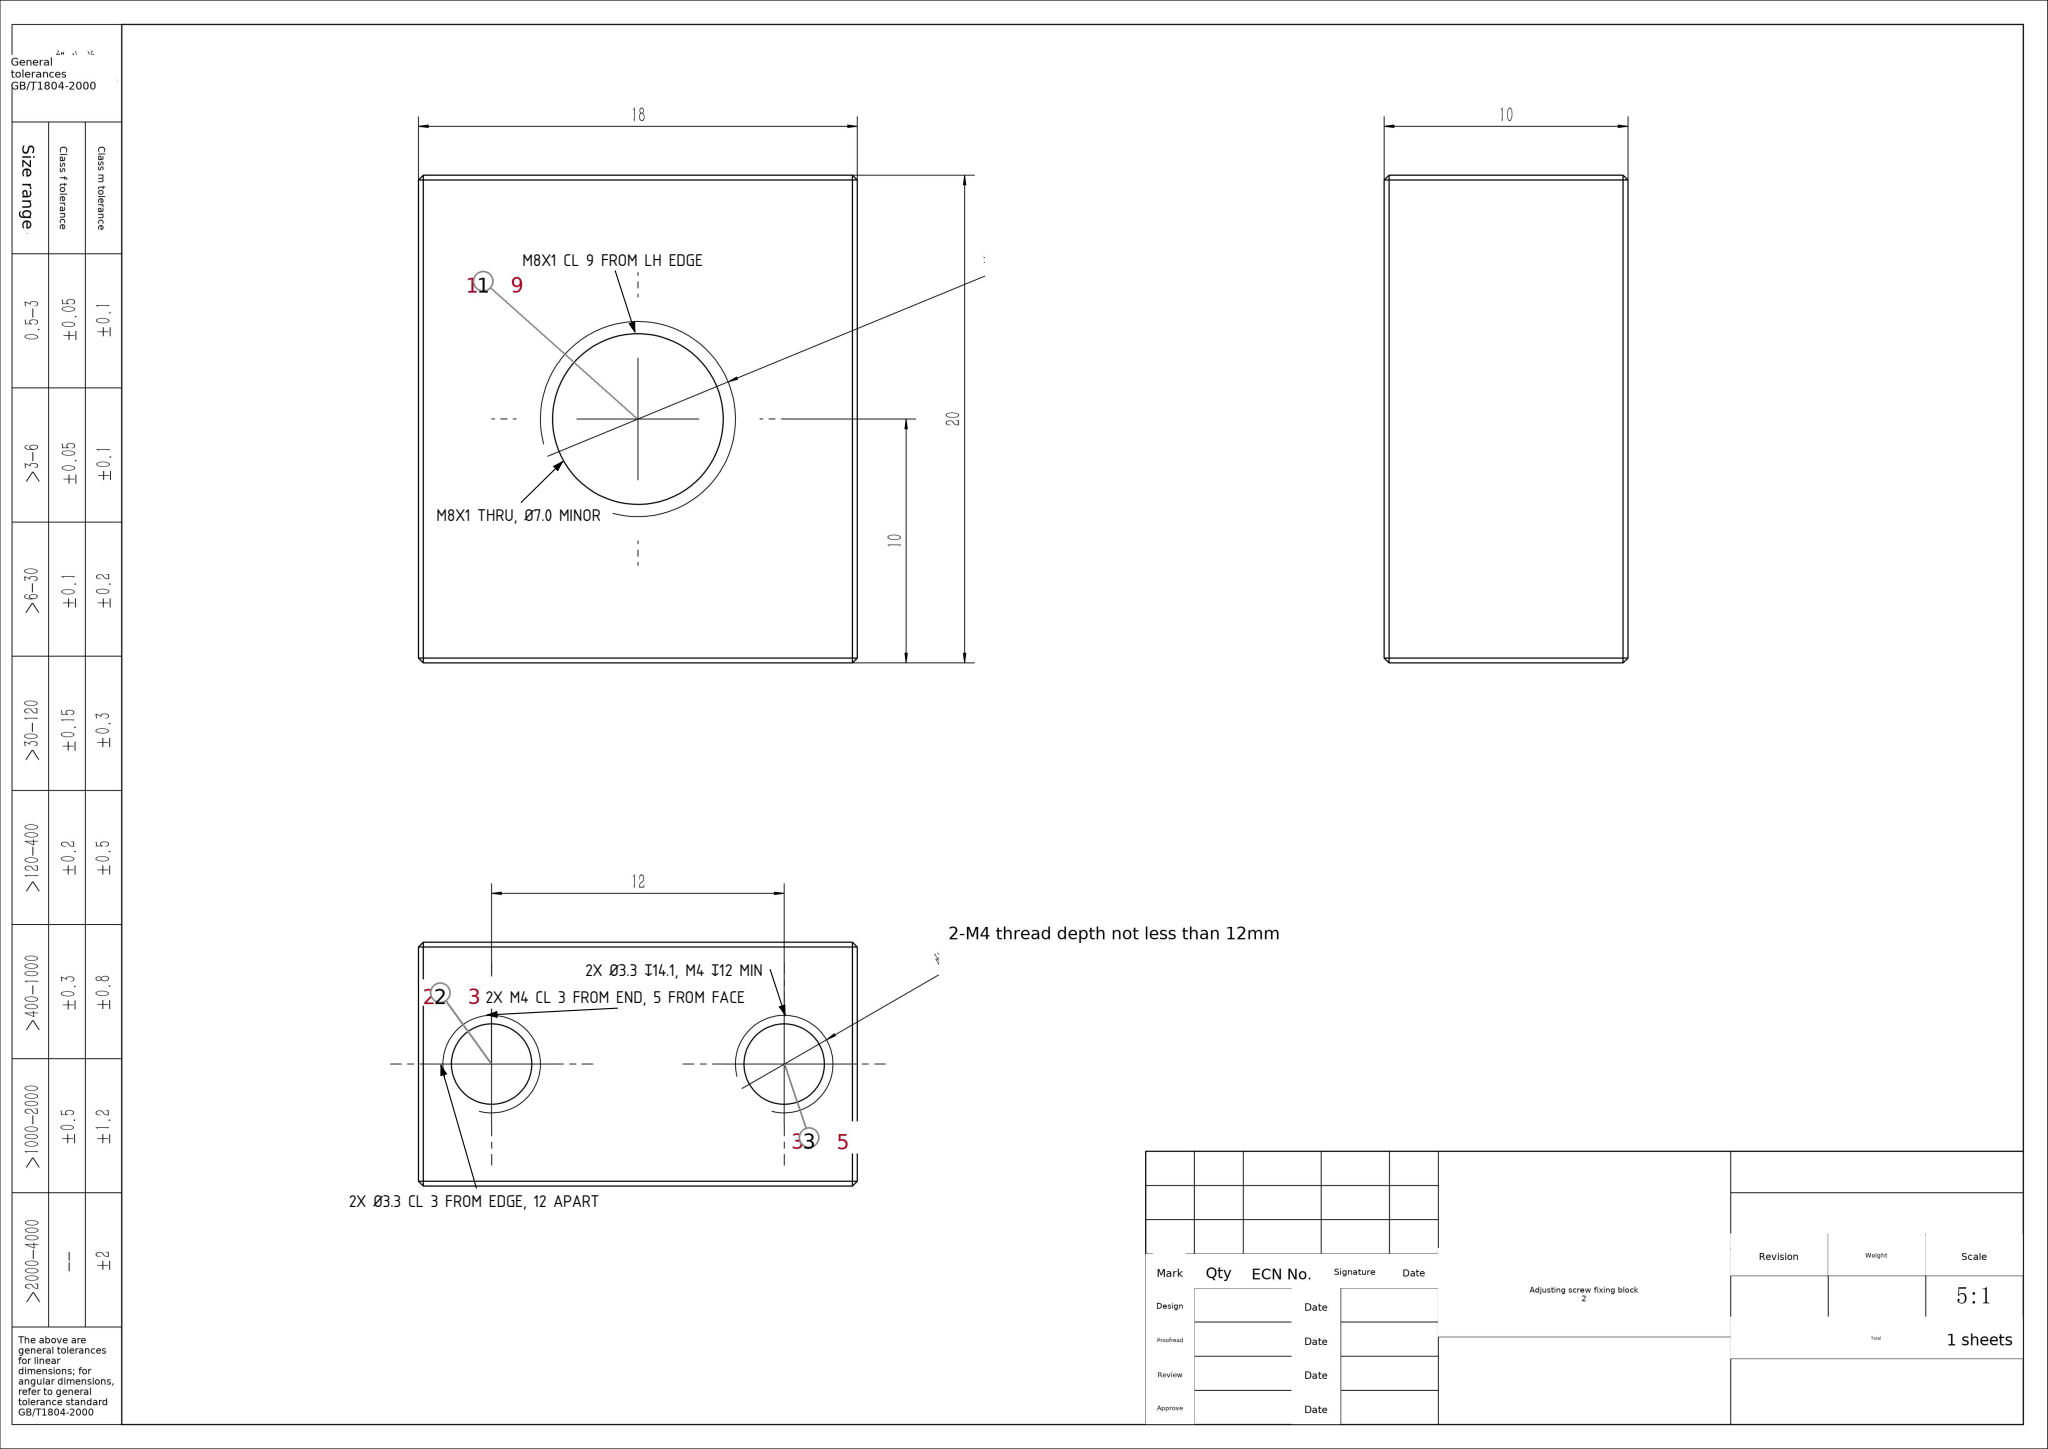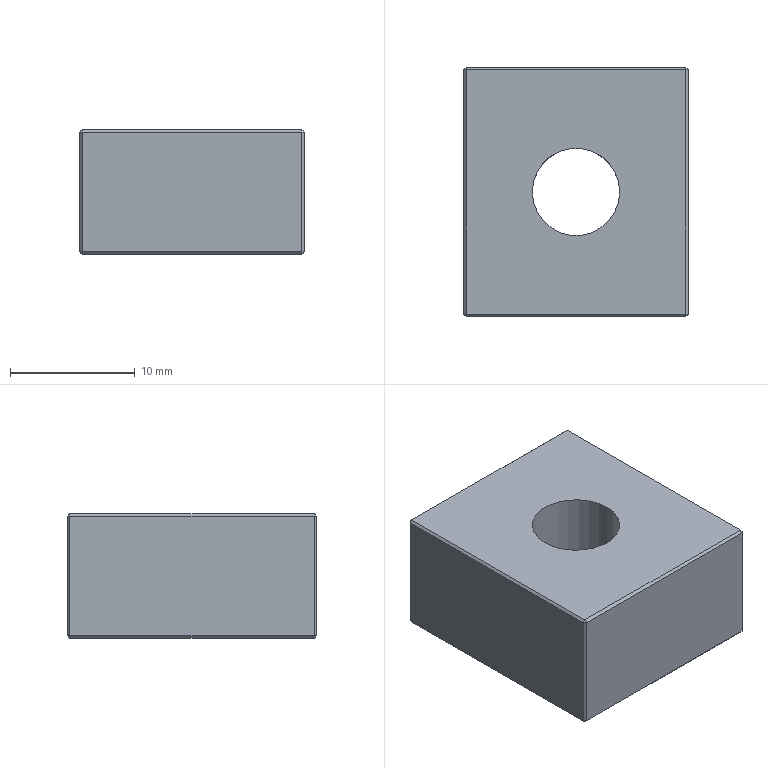Part | SolidWorks | mm | 1 solid | 36 faces | box 18 x 20 x 10 mm | volume 2965 mm3 | plane 26 | cylinder 6 | cone 4 | commonest cylinder face diameters 3.3 x4 7 x2
Drawing notes:
M8X1 HOLE CL 9 FROM LH EDGE (CENTERED IN 18 WIDTH) | from the solid: Ø7.0 z-axis cyl at x=9.0 of 18.0 bbox width
2X M4 HOLE CL 3 FROM EACH END, 5 FROM FACE (CTR OF 10 THK) | from the solid: Ø3.3 y-axis cyls at x=3.0 & 15.0, z=5.0; bbox 18x20x10
2X Ø3.3 DRILL DP 14.1 (118° PT), M4 DP 12 MIN | from the solid: Ø3.3 y-axis cyl length 14.1, cone incl angle 118° ref dia 3.3
CTR HOLE: M8X1 THRU, Ø7.0 MINOR DIA, FULL THD 10 DEEP | from the solid: Ø7.0 cyl, axis Z, pos (9.0,10.0), length 10.0 = full 10 thk; minor dia 7.0 -> M8x1 fine
2X Ø3.3 M4 THD: CL 3.0 FROM LH EDGE, 12 APART, 5.0 FROM FACE | from the solid: Ø3.3 cyls axis Y at x=3.0 and x=15.0, z=5.0; bbox X=18.0 so 15.0 = 3.0 from RH edge
build123d program:
from build123d import *

# Parameters (mm, degrees)
SKETCH1_W             = 18
SKETCH1_H             = 10
BOSS_EXTRUDE1_DEPTH   = 10
M4_TAPPED_HOLE1_D     = 3.3
M4_TAPPED_HOLE1_DEPTH = 14.1
M4_TAPPED_HOLE1_TIP   = 0.9914
M8X1_0_TAPPED_HOLE1_D = 7
CHAMFER1_SIZE         = 0.2


with BuildPart() as part:
    # Sketch1 → Boss-Extrude1 (new, symmetric)
    with BuildSketch(Plane(origin=(0, 0, 0), x_dir=(1, 0, 0), z_dir=(0, 1, 0))):
        Rectangle(SKETCH1_W, SKETCH1_H)
    extrude(amount=BOSS_EXTRUDE1_DEPTH, both=True)

    # M4 Tapped Hole1
    with Locations(Plane(origin=(0, 10, 0), x_dir=(1, 0, 0), z_dir=(0, 1, 0))):
        with Locations((-6, 0), (6, 0)):
            Hole(M4_TAPPED_HOLE1_D / 2, depth=M4_TAPPED_HOLE1_DEPTH)
            with Locations((0, 0, -(M4_TAPPED_HOLE1_DEPTH + M4_TAPPED_HOLE1_TIP / 2))):  # 118° drill point
                Cone(0, M4_TAPPED_HOLE1_D / 2, M4_TAPPED_HOLE1_TIP, mode=Mode.SUBTRACT)

    # M8x1.0 Tapped Hole1 (through all)
    with Locations(Plane.XY.offset(5)):
        with Locations((0, 0)):
            Hole(M8X1_0_TAPPED_HOLE1_D / 2)

    # Chamfer1
    chamfer1_edges = [part.edges().sort_by_distance(p)[0] for p in [
        (-9, 10, 0),
        (0, 10, 5),
        (9, 10, 0),
        (0, -10, 5),
        (-9, -10, 0),
        (0, -10, -5),
        (9, -10, 0),
        (9, 0, 5),
        (-9, 0, 5),
        (-9, 0, -5),
        (9, 0, -5),
        (0, 10, -5),
    ]]
    chamfer(chamfer1_edges, length=CHAMFER1_SIZE)


solid = part.part
STEP:
#1=CARTESIAN_POINT('',(-3.5,0.,-5.));
#2=VERTEX_POINT('',#1);
#3=CARTESIAN_POINT('',(3.5,0.,-5.));
#4=VERTEX_POINT('',#3);
#5=CARTESIAN_POINT('',(0.,0.,-5.));
#6=DIRECTION('',(0.,0.,1.));
#7=DIRECTION('',(1.,0.,0.));
#8=AXIS2_PLACEMENT_3D('',#5,#6,#7);
#9=CIRCLE('',#8,3.5);
#10=EDGE_CURVE('',#2,#4,#9,.T.);
#11=ORIENTED_EDGE('',*,*,#10,.F.);
#12=CARTESIAN_POINT('',(-3.5,0.,5.));
#13=VERTEX_POINT('',#12);
#14=CARTESIAN_POINT('',(-3.5,0.,5.));
#15=DIRECTION('',(0.,0.,1.));
#16=VECTOR('',#15,1000.);
#17=LINE('',#14,#16);
#18=EDGE_CURVE('',#2,#13,#17,.T.);
#19=ORIENTED_EDGE('',*,*,#18,.T.);
#20=CARTESIAN_POINT('',(3.5,0.,5.));
#21=VERTEX_POINT('',#20);
#22=CARTESIAN_POINT('',(0.,0.,5.));
#23=DIRECTION('',(0.,0.,1.));
#24=DIRECTION('',(1.,0.,0.));
#25=AXIS2_PLACEMENT_3D('',#22,#23,#24);
#26=CIRCLE('',#25,3.5);
#27=EDGE_CURVE('',#13,#21,#26,.T.);
#28=ORIENTED_EDGE('',*,*,#27,.T.);
#29=CARTESIAN_POINT('',(3.5,0.,5.));
#30=DIRECTION('',(0.,0.,1.));
#31=VECTOR('',#30,1000.);
#32=LINE('',#29,#31);
#33=EDGE_CURVE('',#4,#21,#32,.T.);
#34=ORIENTED_EDGE('',*,*,#33,.F.);
#35=EDGE_LOOP('',(#11,#19,#28,#34));
#36=FACE_OUTER_BOUND('',#35,.T.);
#37=CARTESIAN_POINT('',(0.,0.,5.));
#38=DIRECTION('',(0.,0.,1.));
#39=DIRECTION('',(1.,0.,0.));
#40=AXIS2_PLACEMENT_3D('',#37,#38,#39);
#41=CYLINDRICAL_SURFACE('',#40,3.5);
#42=ADVANCED_FACE('',(#36),#41,.F.);
#43=CARTESIAN_POINT('',(-6.,-4.1,-1.65));
#44=VERTEX_POINT('',#43);
#45=CARTESIAN_POINT('',(-6.,-4.1,1.65));
#46=VERTEX_POINT('',#45);
#47=CARTESIAN_POINT('',(-6.,-4.1,0.));
#48=DIRECTION('',(0.,1.,0.));
#49=DIRECTION('',(0.,0.,1.));
#50=AXIS2_PLACEMENT_3D('',#47,#48,#49);
#51=CIRCLE('',#50,1.65);
#52=EDGE_CURVE('',#44,#46,#51,.T.);
#53=ORIENTED_EDGE('',*,*,#52,.F.);
#54=CARTESIAN_POINT('',(-6.,10.,-1.65));
#55=VERTEX_POINT('',#54);
#56=CARTESIAN_POINT('',(-6.,10.,-1.65));
#57=DIRECTION('',(0.,1.,0.));
#58=VECTOR('',#57,1000.);
#59=LINE('',#56,#58);
#60=EDGE_CURVE('',#44,#55,#59,.T.);
#61=ORIENTED_EDGE('',*,*,#60,.T.);
#62=CARTESIAN_POINT('',(-6.,10.,1.65));
#63=VERTEX_POINT('',#62);
#64=CARTESIAN_POINT('',(-6.,10.,0.));
#65=DIRECTION('',(0.,1.,0.));
#66=DIRECTION('',(0.,0.,1.));
#67=AXIS2_PLACEMENT_3D('',#64,#65,#66);
#68=CIRCLE('',#67,1.65);
#69=EDGE_CURVE('',#55,#63,#68,.T.);
#70=ORIENTED_EDGE('',*,*,#69,.T.);
#71=CARTESIAN_POINT('',(-6.,10.,1.65));
#72=DIRECTION('',(0.,1.,0.));
#73=VECTOR('',#72,1000.);
#74=LINE('',#71,#73);
#75=EDGE_CURVE('',#46,#63,#74,.T.);
#76=ORIENTED_EDGE('',*,*,#75,.F.);
#77=EDGE_LOOP('',(#53,#61,#70,#76));
#78=FACE_OUTER_BOUND('',#77,.T.);
#79=CARTESIAN_POINT('',(-6.,10.,0.));
#80=DIRECTION('',(0.,1.,0.));
#81=DIRECTION('',(0.,0.,1.));
#82=AXIS2_PLACEMENT_3D('',#79,#80,#81);
#83=CYLINDRICAL_SURFACE('',#82,1.65);
#84=ADVANCED_FACE('',(#78),#83,.F.);
#85=CARTESIAN_POINT('',(-6.,-5.091,0.));
#86=VERTEX_POINT('',#85);
#87=CARTESIAN_POINT('',(-6.,-4.1,1.65));
#88=DIRECTION('',(0.,0.515,0.8572));
#89=VECTOR('',#88,1000.);
#90=LINE('',#87,#89);
#91=EDGE_CURVE('',#86,#46,#90,.T.);
#92=ORIENTED_EDGE('',*,*,#91,.F.);
#93=CARTESIAN_POINT('',(-6.,-4.1,-1.65));
#94=DIRECTION('',(0.,0.515,-0.8572));
#95=VECTOR('',#94,1000.);
#96=LINE('',#93,#95);
#97=EDGE_CURVE('',#86,#44,#96,.T.);
#98=ORIENTED_EDGE('',*,*,#97,.T.);
#99=ORIENTED_EDGE('',*,*,#52,.T.);
#100=EDGE_LOOP('',(#92,#98,#99));
#101=FACE_OUTER_BOUND('',#100,.T.);
#102=CARTESIAN_POINT('',(-6.,-4.1,0.));
#103=DIRECTION('',(0.,1.,0.));
#104=DIRECTION('',(0.,0.,1.));
#105=AXIS2_PLACEMENT_3D('',#102,#103,#104);
#106=CONICAL_SURFACE('',#105,1.65,1.03);
#107=ADVANCED_FACE('',(#101),#106,.F.);
#108=CARTESIAN_POINT('',(6.,-4.1,-1.65));
#109=VERTEX_POINT('',#108);
#110=CARTESIAN_POINT('',(6.,-4.1,1.65));
#111=VERTEX_POINT('',#110);
#112=CARTESIAN_POINT('',(6.,-4.1,-0.));
#113=DIRECTION('',(0.,1.,0.));
#114=DIRECTION('',(0.,0.,1.));
#115=AXIS2_PLACEMENT_3D('',#112,#113,#114);
#116=CIRCLE('',#115,1.65);
#117=EDGE_CURVE('',#109,#111,#116,.T.);
#118=ORIENTED_EDGE('',*,*,#117,.F.);
#119=CARTESIAN_POINT('',(6.,10.,-1.65));
#120=VERTEX_POINT('',#119);
#121=CARTESIAN_POINT('',(6.,10.,-1.65));
#122=DIRECTION('',(0.,1.,0.));
#123=VECTOR('',#122,1000.);
#124=LINE('',#121,#123);
#125=EDGE_CURVE('',#109,#120,#124,.T.);
#126=ORIENTED_EDGE('',*,*,#125,.T.);
#127=CARTESIAN_POINT('',(6.,10.,1.65));
#128=VERTEX_POINT('',#127);
#129=CARTESIAN_POINT('',(6.,10.,-0.));
#130=DIRECTION('',(0.,1.,0.));
#131=DIRECTION('',(0.,0.,1.));
#132=AXIS2_PLACEMENT_3D('',#129,#130,#131);
#133=CIRCLE('',#132,1.65);
#134=EDGE_CURVE('',#120,#128,#133,.T.);
#135=ORIENTED_EDGE('',*,*,#134,.T.);
#136=CARTESIAN_POINT('',(6.,10.,1.65));
#137=DIRECTION('',(0.,1.,0.));
#138=VECTOR('',#137,1000.);
#139=LINE('',#136,#138);
#140=EDGE_CURVE('',#111,#128,#139,.T.);
#141=ORIENTED_EDGE('',*,*,#140,.F.);
#142=EDGE_LOOP('',(#118,#126,#135,#141));
#143=FACE_OUTER_BOUND('',#142,.T.);
#144=CARTESIAN_POINT('',(6.,10.,-0.));
#145=DIRECTION('',(0.,1.,0.));
#146=DIRECTION('',(0.,0.,1.));
#147=AXIS2_PLACEMENT_3D('',#144,#145,#146);
#148=CYLINDRICAL_SURFACE('',#147,1.65);
#149=ADVANCED_FACE('',(#143),#148,.F.);
#150=CARTESIAN_POINT('',(6.,-5.091,-0.));
#151=VERTEX_POINT('',#150);
#152=CARTESIAN_POINT('',(6.,-4.1,1.65));
#153=DIRECTION('',(0.,0.515,0.8572));
#154=VECTOR('',#153,1000.);
#155=LINE('',#152,#154);
#156=EDGE_CURVE('',#151,#111,#155,.T.);
#157=ORIENTED_EDGE('',*,*,#156,.F.);
#158=CARTESIAN_POINT('',(6.,-4.1,-1.65));
#159=DIRECTION('',(0.,0.515,-0.8572));
#160=VECTOR('',#159,1000.);
#161=LINE('',#158,#160);
#162=EDGE_CURVE('',#151,#109,#161,.T.);
#163=ORIENTED_EDGE('',*,*,#162,.T.);
#164=ORIENTED_EDGE('',*,*,#117,.T.);
#165=EDGE_LOOP('',(#157,#163,#164));
#166=FACE_OUTER_BOUND('',#165,.T.);
#167=CARTESIAN_POINT('',(6.,-4.1,-0.));
#168=DIRECTION('',(0.,1.,0.));
#169=DIRECTION('',(0.,0.,1.));
#170=AXIS2_PLACEMENT_3D('',#167,#168,#169);
#171=CONICAL_SURFACE('',#170,1.65,1.03);
#172=ADVANCED_FACE('',(#166),#171,.F.);
#173=CARTESIAN_POINT('',(9.,9.8,-4.8));
#174=VERTEX_POINT('',#173);
#175=CARTESIAN_POINT('',(9.,9.8,4.8));
#176=VERTEX_POINT('',#175);
#177=CARTESIAN_POINT('',(9.,9.8,5.));
#178=DIRECTION('',(0.,0.,1.));
#179=VECTOR('',#178,1000.);
#180=LINE('',#177,#179);
#181=EDGE_CURVE('',#174,#176,#180,.T.);
#182=ORIENTED_EDGE('',*,*,#181,.T.);
#183=CARTESIAN_POINT('',(9.,-9.8,4.8));
#184=VERTEX_POINT('',#183);
#185=CARTESIAN_POINT('',(9.,10.,4.8));
#186=DIRECTION('',(0.,-1.,0.));
#187=VECTOR('',#186,1000.);
#188=LINE('',#185,#187);
#189=EDGE_CURVE('',#176,#184,#188,.T.);
#190=ORIENTED_EDGE('',*,*,#189,.T.);
#191=CARTESIAN_POINT('',(9.,-9.8,-4.8));
#192=VERTEX_POINT('',#191);
#193=CARTESIAN_POINT('',(9.,-9.8,-5.));
#194=DIRECTION('',(0.,0.,-1.));
#195=VECTOR('',#194,1000.);
#196=LINE('',#193,#195);
#197=EDGE_CURVE('',#184,#192,#196,.T.);
#198=ORIENTED_EDGE('',*,*,#197,.T.);
#199=CARTESIAN_POINT('',(9.,10.,-4.8));
#200=DIRECTION('',(0.,1.,0.));
#201=VECTOR('',#200,1000.);
#202=LINE('',#199,#201);
#203=EDGE_CURVE('',#192,#174,#202,.T.);
#204=ORIENTED_EDGE('',*,*,#203,.T.);
#205=EDGE_LOOP('',(#182,#190,#198,#204));
#206=FACE_OUTER_BOUND('',#205,.T.);
#207=CARTESIAN_POINT('',(9.,10.,-5.));
#208=DIRECTION('',(-1.,0.,0.));
#209=DIRECTION('',(0.,0.,1.));
#210=AXIS2_PLACEMENT_3D('',#207,#208,#209);
#211=PLANE('',#210);
#212=ADVANCED_FACE('',(#206),#211,.F.);
#213=CARTESIAN_POINT('',(8.8,-9.8,-5.));
#214=VERTEX_POINT('',#213);
#215=CARTESIAN_POINT('',(-8.8,-9.8,-5.));
#216=VERTEX_POINT('',#215);
#217=CARTESIAN_POINT('',(-9.,-9.8,-5.));
#218=DIRECTION('',(-1.,0.,0.));
#219=VECTOR('',#218,1000.);
#220=LINE('',#217,#219);
#221=EDGE_CURVE('',#214,#216,#220,.T.);
#222=ORIENTED_EDGE('',*,*,#221,.T.);
#223=CARTESIAN_POINT('',(-8.8,9.8,-5.));
#224=VERTEX_POINT('',#223);
#225=CARTESIAN_POINT('',(-8.8,10.,-5.));
#226=DIRECTION('',(0.,1.,0.));
#227=VECTOR('',#226,1000.);
#228=LINE('',#225,#227);
#229=EDGE_CURVE('',#216,#224,#228,.T.);
#230=ORIENTED_EDGE('',*,*,#229,.T.);
#231=CARTESIAN_POINT('',(8.8,9.8,-5.));
#232=VERTEX_POINT('',#231);
#233=CARTESIAN_POINT('',(9.,9.8,-5.));
#234=DIRECTION('',(1.,0.,0.));
#235=VECTOR('',#234,1000.);
#236=LINE('',#233,#235);
#237=EDGE_CURVE('',#224,#232,#236,.T.);
#238=ORIENTED_EDGE('',*,*,#237,.T.);
#239=CARTESIAN_POINT('',(8.8,10.,-5.));
#240=DIRECTION('',(0.,-1.,0.));
#241=VECTOR('',#240,1000.);
#242=LINE('',#239,#241);
#243=EDGE_CURVE('',#232,#214,#242,.T.);
#244=ORIENTED_EDGE('',*,*,#243,.T.);
#245=EDGE_LOOP('',(#222,#230,#238,#244));
#246=FACE_OUTER_BOUND('',#245,.T.);
#247=CARTESIAN_POINT('',(0.,0.,-5.));
#248=DIRECTION('',(0.,0.,1.));
#249=DIRECTION('',(1.,0.,0.));
#250=AXIS2_PLACEMENT_3D('',#247,#248,#249);
#251=CIRCLE('',#250,3.5);
#252=EDGE_CURVE('',#4,#2,#251,.T.);
#253=ORIENTED_EDGE('',*,*,#252,.T.);
#254=ORIENTED_EDGE('',*,*,#10,.T.);
#255=EDGE_LOOP('',(#253,#254));
#256=FACE_BOUND('',#255,.T.);
#257=CARTESIAN_POINT('',(-9.,10.,-5.));
#258=DIRECTION('',(0.,0.,1.));
#259=DIRECTION('',(1.,0.,0.));
#260=AXIS2_PLACEMENT_3D('',#257,#258,#259);
#261=PLANE('',#260);
#262=ADVANCED_FACE('',(#246,#256),#261,.F.);
#263=CARTESIAN_POINT('',(-9.,9.8,4.8));
#264=VERTEX_POINT('',#263);
#265=CARTESIAN_POINT('',(-9.,9.8,-4.8));
#266=VERTEX_POINT('',#265);
#267=CARTESIAN_POINT('',(-9.,9.8,-5.));
#268=DIRECTION('',(0.,0.,-1.));
#269=VECTOR('',#268,1000.);
#270=LINE('',#267,#269);
#271=EDGE_CURVE('',#264,#266,#270,.T.);
#272=ORIENTED_EDGE('',*,*,#271,.T.);
#273=CARTESIAN_POINT('',(-9.,-9.8,-4.8));
#274=VERTEX_POINT('',#273);
#275=CARTESIAN_POINT('',(-9.,10.,-4.8));
#276=DIRECTION('',(0.,-1.,0.));
#277=VECTOR('',#276,1000.);
#278=LINE('',#275,#277);
#279=EDGE_CURVE('',#266,#274,#278,.T.);
#280=ORIENTED_EDGE('',*,*,#279,.T.);
#281=CARTESIAN_POINT('',(-9.,-9.8,4.8));
#282=VERTEX_POINT('',#281);
#283=CARTESIAN_POINT('',(-9.,-9.8,-5.));
#284=DIRECTION('',(0.,0.,1.));
#285=VECTOR('',#284,1000.);
#286=LINE('',#283,#285);
#287=EDGE_CURVE('',#274,#282,#286,.T.);
#288=ORIENTED_EDGE('',*,*,#287,.T.);
#289=CARTESIAN_POINT('',(-9.,10.,4.8));
#290=DIRECTION('',(0.,1.,0.));
#291=VECTOR('',#290,1000.);
#292=LINE('',#289,#291);
#293=EDGE_CURVE('',#282,#264,#292,.T.);
#294=ORIENTED_EDGE('',*,*,#293,.T.);
#295=EDGE_LOOP('',(#272,#280,#288,#294));
#296=FACE_OUTER_BOUND('',#295,.T.);
#297=CARTESIAN_POINT('',(-9.,10.,-5.));
#298=DIRECTION('',(1.,0.,0.));
#299=DIRECTION('',(0.,0.,-1.));
#300=AXIS2_PLACEMENT_3D('',#297,#298,#299);
#301=PLANE('',#300);
#302=ADVANCED_FACE('',(#296),#301,.F.);
#303=CARTESIAN_POINT('',(-8.8,9.8,5.));
#304=VERTEX_POINT('',#303);
#305=CARTESIAN_POINT('',(-8.8,-9.8,5.));
#306=VERTEX_POINT('',#305);
#307=CARTESIAN_POINT('',(-8.8,10.,5.));
#308=DIRECTION('',(0.,-1.,0.));
#309=VECTOR('',#308,1000.);
#310=LINE('',#307,#309);
#311=EDGE_CURVE('',#304,#306,#310,.T.);
#312=ORIENTED_EDGE('',*,*,#311,.T.);
#313=CARTESIAN_POINT('',(8.8,-9.8,5.));
#314=VERTEX_POINT('',#313);
#315=CARTESIAN_POINT('',(-9.,-9.8,5.));
#316=DIRECTION('',(1.,0.,0.));
#317=VECTOR('',#316,1000.);
#318=LINE('',#315,#317);
#319=EDGE_CURVE('',#306,#314,#318,.T.);
#320=ORIENTED_EDGE('',*,*,#319,.T.);
#321=CARTESIAN_POINT('',(8.8,9.8,5.));
#322=VERTEX_POINT('',#321);
#323=CARTESIAN_POINT('',(8.8,10.,5.));
#324=DIRECTION('',(0.,1.,0.));
#325=VECTOR('',#324,1000.);
#326=LINE('',#323,#325);
#327=EDGE_CURVE('',#314,#322,#326,.T.);
#328=ORIENTED_EDGE('',*,*,#327,.T.);
#329=CARTESIAN_POINT('',(-9.,9.8,5.));
#330=DIRECTION('',(-1.,0.,0.));
#331=VECTOR('',#330,1000.);
#332=LINE('',#329,#331);
#333=EDGE_CURVE('',#322,#304,#332,.T.);
#334=ORIENTED_EDGE('',*,*,#333,.T.);
#335=EDGE_LOOP('',(#312,#320,#328,#334));
#336=FACE_OUTER_BOUND('',#335,.T.);
#337=CARTESIAN_POINT('',(0.,0.,5.));
#338=DIRECTION('',(0.,0.,1.));
#339=DIRECTION('',(1.,0.,0.));
#340=AXIS2_PLACEMENT_3D('',#337,#338,#339);
#341=CIRCLE('',#340,3.5);
#342=EDGE_CURVE('',#21,#13,#341,.T.);
#343=ORIENTED_EDGE('',*,*,#342,.F.);
#344=ORIENTED_EDGE('',*,*,#27,.F.);
#345=EDGE_LOOP('',(#343,#344));
#346=FACE_BOUND('',#345,.T.);
#347=CARTESIAN_POINT('',(-9.,10.,5.));
#348=DIRECTION('',(0.,0.,-1.));
#349=DIRECTION('',(-1.,0.,0.));
#350=AXIS2_PLACEMENT_3D('',#347,#348,#349);
#351=PLANE('',#350);
#352=ADVANCED_FACE('',(#336,#346),#351,.F.);
#353=CARTESIAN_POINT('',(8.8,10.,-4.8));
#354=VERTEX_POINT('',#353);
#355=CARTESIAN_POINT('',(-8.8,10.,-4.8));
#356=VERTEX_POINT('',#355);
#357=CARTESIAN_POINT('',(-9.,10.,-4.8));
#358=DIRECTION('',(-1.,0.,0.));
#359=VECTOR('',#358,1000.);
#360=LINE('',#357,#359);
#361=EDGE_CURVE('',#354,#356,#360,.T.);
#362=ORIENTED_EDGE('',*,*,#361,.T.);
#363=CARTESIAN_POINT('',(-8.8,10.,4.8));
#364=VERTEX_POINT('',#363);
#365=CARTESIAN_POINT('',(-8.8,10.,5.));
#366=DIRECTION('',(0.,0.,1.));
#367=VECTOR('',#366,1000.);
#368=LINE('',#365,#367);
#369=EDGE_CURVE('',#356,#364,#368,.T.);
#370=ORIENTED_EDGE('',*,*,#369,.T.);
#371=CARTESIAN_POINT('',(8.8,10.,4.8));
#372=VERTEX_POINT('',#371);
#373=CARTESIAN_POINT('',(9.,10.,4.8));
#374=DIRECTION('',(1.,0.,0.));
#375=VECTOR('',#374,1000.);
#376=LINE('',#373,#375);
#377=EDGE_CURVE('',#364,#372,#376,.T.);
#378=ORIENTED_EDGE('',*,*,#377,.T.);
#379=CARTESIAN_POINT('',(8.8,10.,-5.));
#380=DIRECTION('',(0.,0.,-1.));
#381=VECTOR('',#380,1000.);
#382=LINE('',#379,#381);
#383=EDGE_CURVE('',#372,#354,#382,.T.);
#384=ORIENTED_EDGE('',*,*,#383,.T.);
#385=EDGE_LOOP('',(#362,#370,#378,#384));
#386=FACE_OUTER_BOUND('',#385,.T.);
#387=CARTESIAN_POINT('',(-6.,10.,0.));
#388=DIRECTION('',(0.,1.,0.));
#389=DIRECTION('',(0.,0.,1.));
#390=AXIS2_PLACEMENT_3D('',#387,#388,#389);
#391=CIRCLE('',#390,1.65);
#392=EDGE_CURVE('',#63,#55,#391,.T.);
#393=ORIENTED_EDGE('',*,*,#392,.F.);
#394=ORIENTED_EDGE('',*,*,#69,.F.);
#395=EDGE_LOOP('',(#393,#394));
#396=FACE_BOUND('',#395,.T.);
#397=CARTESIAN_POINT('',(6.,10.,-0.));
#398=DIRECTION('',(0.,1.,0.));
#399=DIRECTION('',(0.,0.,1.));
#400=AXIS2_PLACEMENT_3D('',#397,#398,#399);
#401=CIRCLE('',#400,1.65);
#402=EDGE_CURVE('',#128,#120,#401,.T.);
#403=ORIENTED_EDGE('',*,*,#402,.F.);
#404=ORIENTED_EDGE('',*,*,#134,.F.);
#405=EDGE_LOOP('',(#403,#404));
#406=FACE_BOUND('',#405,.T.);
#407=CARTESIAN_POINT('',(0.,10.,0.));
#408=DIRECTION('',(0.,1.,0.));
#409=DIRECTION('',(0.,0.,1.));
#410=AXIS2_PLACEMENT_3D('',#407,#408,#409);
#411=PLANE('',#410);
#412=ADVANCED_FACE('',(#386,#396,#406),#411,.T.);
#413=CARTESIAN_POINT('',(8.8,-10.,4.8));
#414=VERTEX_POINT('',#413);
#415=CARTESIAN_POINT('',(-8.8,-10.,4.8));
#416=VERTEX_POINT('',#415);
#417=CARTESIAN_POINT('',(0.,-10.,4.8));
#418=DIRECTION('',(-1.,0.,0.));
#419=VECTOR('',#418,1000.);
#420=LINE('',#417,#419);
#421=EDGE_CURVE('',#414,#416,#420,.T.);
#422=ORIENTED_EDGE('',*,*,#421,.T.);
#423=CARTESIAN_POINT('',(-8.8,-10.,-4.8));
#424=VERTEX_POINT('',#423);
#425=CARTESIAN_POINT('',(-8.8,-10.,0.));
#426=DIRECTION('',(0.,0.,-1.));
#427=VECTOR('',#426,1000.);
#428=LINE('',#425,#427);
#429=EDGE_CURVE('',#416,#424,#428,.T.);
#430=ORIENTED_EDGE('',*,*,#429,.T.);
#431=CARTESIAN_POINT('',(8.8,-10.,-4.8));
#432=VERTEX_POINT('',#431);
#433=CARTESIAN_POINT('',(0.,-10.,-4.8));
#434=DIRECTION('',(1.,0.,0.));
#435=VECTOR('',#434,1000.);
#436=LINE('',#433,#435);
#437=EDGE_CURVE('',#424,#432,#436,.T.);
#438=ORIENTED_EDGE('',*,*,#437,.T.);
#439=CARTESIAN_POINT('',(8.8,-10.,0.));
#440=DIRECTION('',(0.,0.,1.));
#441=VECTOR('',#440,1000.);
#442=LINE('',#439,#441);
#443=EDGE_CURVE('',#432,#414,#442,.T.);
#444=ORIENTED_EDGE('',*,*,#443,.T.);
#445=EDGE_LOOP('',(#422,#430,#438,#444));
#446=FACE_OUTER_BOUND('',#445,.T.);
#447=CARTESIAN_POINT('',(0.,-10.,0.));
#448=DIRECTION('',(0.,1.,0.));
#449=DIRECTION('',(0.,0.,1.));
#450=AXIS2_PLACEMENT_3D('',#447,#448,#449);
#451=PLANE('',#450);
#452=ADVANCED_FACE('',(#446),#451,.F.);
#453=ORIENTED_EDGE('',*,*,#162,.F.);
#454=ORIENTED_EDGE('',*,*,#156,.T.);
#455=CARTESIAN_POINT('',(6.,-4.1,-0.));
#456=DIRECTION('',(0.,1.,0.));
#457=DIRECTION('',(0.,0.,1.));
#458=AXIS2_PLACEMENT_3D('',#455,#456,#457);
#459=CIRCLE('',#458,1.65);
#460=EDGE_CURVE('',#111,#109,#459,.T.);
#461=ORIENTED_EDGE('',*,*,#460,.T.);
#462=EDGE_LOOP('',(#453,#454,#461));
#463=FACE_OUTER_BOUND('',#462,.T.);
#464=CARTESIAN_POINT('',(6.,-4.1,-0.));
#465=DIRECTION('',(0.,1.,0.));
#466=DIRECTION('',(0.,0.,1.));
#467=AXIS2_PLACEMENT_3D('',#464,#465,#466);
#468=CONICAL_SURFACE('',#467,1.65,1.03);
#469=ADVANCED_FACE('',(#463),#468,.F.);
#470=ORIENTED_EDGE('',*,*,#125,.F.);
#471=ORIENTED_EDGE('',*,*,#460,.F.);
#472=ORIENTED_EDGE('',*,*,#140,.T.);
#473=ORIENTED_EDGE('',*,*,#402,.T.);
#474=EDGE_LOOP('',(#470,#471,#472,#473));
#475=FACE_OUTER_BOUND('',#474,.T.);
#476=CARTESIAN_POINT('',(6.,10.,-0.));
#477=DIRECTION('',(0.,1.,0.));
#478=DIRECTION('',(0.,0.,1.));
#479=AXIS2_PLACEMENT_3D('',#476,#477,#478);
#480=CYLINDRICAL_SURFACE('',#479,1.65);
#481=ADVANCED_FACE('',(#475),#480,.F.);
#482=ORIENTED_EDGE('',*,*,#97,.F.);
#483=ORIENTED_EDGE('',*,*,#91,.T.);
#484=CARTESIAN_POINT('',(-6.,-4.1,0.));
#485=DIRECTION('',(0.,1.,0.));
#486=DIRECTION('',(0.,0.,1.));
#487=AXIS2_PLACEMENT_3D('',#484,#485,#486);
#488=CIRCLE('',#487,1.65);
#489=EDGE_CURVE('',#46,#44,#488,.T.);
#490=ORIENTED_EDGE('',*,*,#489,.T.);
#491=EDGE_LOOP('',(#482,#483,#490));
#492=FACE_OUTER_BOUND('',#491,.T.);
#493=CARTESIAN_POINT('',(-6.,-4.1,0.));
#494=DIRECTION('',(0.,1.,0.));
#495=DIRECTION('',(0.,0.,1.));
#496=AXIS2_PLACEMENT_3D('',#493,#494,#495);
#497=CONICAL_SURFACE('',#496,1.65,1.03);
#498=ADVANCED_FACE('',(#492),#497,.F.);
#499=ORIENTED_EDGE('',*,*,#60,.F.);
#500=ORIENTED_EDGE('',*,*,#489,.F.);
#501=ORIENTED_EDGE('',*,*,#75,.T.);
#502=ORIENTED_EDGE('',*,*,#392,.T.);
#503=EDGE_LOOP('',(#499,#500,#501,#502));
#504=FACE_OUTER_BOUND('',#503,.T.);
#505=CARTESIAN_POINT('',(-6.,10.,0.));
#506=DIRECTION('',(0.,1.,0.));
#507=DIRECTION('',(0.,0.,1.));
#508=AXIS2_PLACEMENT_3D('',#505,#506,#507);
#509=CYLINDRICAL_SURFACE('',#508,1.65);
#510=ADVANCED_FACE('',(#504),#509,.F.);
#511=ORIENTED_EDGE('',*,*,#18,.F.);
#512=ORIENTED_EDGE('',*,*,#252,.F.);
#513=ORIENTED_EDGE('',*,*,#33,.T.);
#514=ORIENTED_EDGE('',*,*,#342,.T.);
#515=EDGE_LOOP('',(#511,#512,#513,#514));
#516=FACE_OUTER_BOUND('',#515,.T.);
#517=CARTESIAN_POINT('',(0.,0.,5.));
#518=DIRECTION('',(0.,0.,1.));
#519=DIRECTION('',(1.,0.,0.));
#520=AXIS2_PLACEMENT_3D('',#517,#518,#519);
#521=CYLINDRICAL_SURFACE('',#520,3.5);
#522=ADVANCED_FACE('',(#516),#521,.F.);
#523=CARTESIAN_POINT('',(8.8,9.8,5.));
#524=DIRECTION('',(0.7071,0.,-0.7071));
#525=VECTOR('',#524,1000.);
#526=LINE('',#523,#525);
#527=EDGE_CURVE('',#322,#176,#526,.T.);
#528=ORIENTED_EDGE('',*,*,#527,.F.);
#529=ORIENTED_EDGE('',*,*,#327,.F.);
#530=CARTESIAN_POINT('',(9.,-9.8,4.8));
#531=DIRECTION('',(-0.7071,0.,0.7071));
#532=VECTOR('',#531,1000.);
#533=LINE('',#530,#532);
#534=EDGE_CURVE('',#184,#314,#533,.T.);
#535=ORIENTED_EDGE('',*,*,#534,.F.);
#536=ORIENTED_EDGE('',*,*,#189,.F.);
#537=EDGE_LOOP('',(#528,#529,#535,#536));
#538=FACE_OUTER_BOUND('',#537,.T.);
#539=CARTESIAN_POINT('',(9.,10.,4.8));
#540=DIRECTION('',(-0.7071,0.,-0.7071));
#541=DIRECTION('',(0.,-1.,0.));
#542=AXIS2_PLACEMENT_3D('',#539,#540,#541);
#543=PLANE('',#542);
#544=ADVANCED_FACE('',(#538),#543,.F.);
#545=CARTESIAN_POINT('',(8.8,9.8,5.));
#546=DIRECTION('',(0.,0.7071,-0.7071));
#547=VECTOR('',#546,1000.);
#548=LINE('',#545,#547);
#549=EDGE_CURVE('',#322,#372,#548,.T.);
#550=ORIENTED_EDGE('',*,*,#549,.F.);
#551=ORIENTED_EDGE('',*,*,#527,.T.);
#552=CARTESIAN_POINT('',(8.9,9.9,4.8));
#553=DIRECTION('',(0.7071,-0.7071,0.));
#554=VECTOR('',#553,1000.);
#555=LINE('',#552,#554);
#556=EDGE_CURVE('',#372,#176,#555,.T.);
#557=ORIENTED_EDGE('',*,*,#556,.F.);
#558=EDGE_LOOP('',(#550,#551,#557));
#559=FACE_OUTER_BOUND('',#558,.T.);
#560=CARTESIAN_POINT('',(8.8,9.8,5.));
#561=DIRECTION('',(0.5774,0.5774,0.5774));
#562=DIRECTION('',(0.7071,0.,-0.7071));
#563=AXIS2_PLACEMENT_3D('',#560,#561,#562);
#564=PLANE('',#563);
#565=ADVANCED_FACE('',(#559),#564,.T.);
#566=CARTESIAN_POINT('',(9.,-9.8,4.8));
#567=DIRECTION('',(-0.7071,-0.7071,0.));
#568=VECTOR('',#567,1000.);
#569=LINE('',#566,#568);
#570=EDGE_CURVE('',#184,#414,#569,.T.);
#571=ORIENTED_EDGE('',*,*,#570,.F.);
#572=ORIENTED_EDGE('',*,*,#534,.T.);
#573=CARTESIAN_POINT('',(8.8,-9.9,4.9));
#574=DIRECTION('',(0.,0.7071,0.7071));
#575=VECTOR('',#574,1000.);
#576=LINE('',#573,#575);
#577=EDGE_CURVE('',#414,#314,#576,.T.);
#578=ORIENTED_EDGE('',*,*,#577,.F.);
#579=EDGE_LOOP('',(#571,#572,#578));
#580=FACE_OUTER_BOUND('',#579,.T.);
#581=CARTESIAN_POINT('',(9.,-9.8,4.8));
#582=DIRECTION('',(0.5774,-0.5774,0.5774));
#583=DIRECTION('',(0.7071,0.,-0.7071));
#584=AXIS2_PLACEMENT_3D('',#581,#582,#583);
#585=PLANE('',#584);
#586=ADVANCED_FACE('',(#580),#585,.T.);
#587=ORIENTED_EDGE('',*,*,#556,.T.);
#588=ORIENTED_EDGE('',*,*,#181,.F.);
#589=CARTESIAN_POINT('',(9.,9.8,-4.8));
#590=DIRECTION('',(0.7071,-0.7071,0.));
#591=VECTOR('',#590,1000.);
#592=LINE('',#589,#591);
#593=EDGE_CURVE('',#354,#174,#592,.T.);
#594=ORIENTED_EDGE('',*,*,#593,.F.);
#595=ORIENTED_EDGE('',*,*,#383,.F.);
#596=EDGE_LOOP('',(#587,#588,#594,#595));
#597=FACE_OUTER_BOUND('',#596,.T.);
#598=CARTESIAN_POINT('',(8.8,10.,0.));
#599=DIRECTION('',(0.7071,0.7071,0.));
#600=DIRECTION('',(0.,0.,1.));
#601=AXIS2_PLACEMENT_3D('',#598,#599,#600);
#602=PLANE('',#601);
#603=ADVANCED_FACE('',(#597),#602,.T.);
#604=ORIENTED_EDGE('',*,*,#549,.T.);
#605=ORIENTED_EDGE('',*,*,#377,.F.);
#606=CARTESIAN_POINT('',(-8.8,10.,4.8));
#607=DIRECTION('',(0.,0.7071,-0.7071));
#608=VECTOR('',#607,1000.);
#609=LINE('',#606,#608);
#610=EDGE_CURVE('',#304,#364,#609,.T.);
#611=ORIENTED_EDGE('',*,*,#610,.F.);
#612=ORIENTED_EDGE('',*,*,#333,.F.);
#613=EDGE_LOOP('',(#604,#605,#611,#612));
#614=FACE_OUTER_BOUND('',#613,.T.);
#615=CARTESIAN_POINT('',(0.,10.,4.8));
#616=DIRECTION('',(0.,0.7071,0.7071));
#617=DIRECTION('',(-1.,0.,0.));
#618=AXIS2_PLACEMENT_3D('',#615,#616,#617);
#619=PLANE('',#618);
#620=ADVANCED_FACE('',(#614),#619,.T.);
#621=CARTESIAN_POINT('',(-8.8,-9.8,5.));
#622=DIRECTION('',(-0.7071,0.,-0.7071));
#623=VECTOR('',#622,1000.);
#624=LINE('',#621,#623);
#625=EDGE_CURVE('',#306,#282,#624,.T.);
#626=ORIENTED_EDGE('',*,*,#625,.F.);
#627=ORIENTED_EDGE('',*,*,#311,.F.);
#628=CARTESIAN_POINT('',(-8.9,9.8,4.9));
#629=DIRECTION('',(0.7071,0.,0.7071));
#630=VECTOR('',#629,1000.);
#631=LINE('',#628,#630);
#632=EDGE_CURVE('',#264,#304,#631,.T.);
#633=ORIENTED_EDGE('',*,*,#632,.F.);
#634=ORIENTED_EDGE('',*,*,#293,.F.);
#635=EDGE_LOOP('',(#626,#627,#633,#634));
#636=FACE_OUTER_BOUND('',#635,.T.);
#637=CARTESIAN_POINT('',(-8.8,10.,5.));
#638=DIRECTION('',(0.7071,0.,-0.7071));
#639=DIRECTION('',(0.,-1.,0.));
#640=AXIS2_PLACEMENT_3D('',#637,#638,#639);
#641=PLANE('',#640);
#642=ADVANCED_FACE('',(#636),#641,.F.);
#643=ORIENTED_EDGE('',*,*,#577,.T.);
#644=ORIENTED_EDGE('',*,*,#319,.F.);
#645=CARTESIAN_POINT('',(-8.8,-9.8,5.));
#646=DIRECTION('',(0.,0.7071,0.7071));
#647=VECTOR('',#646,1000.);
#648=LINE('',#645,#647);
#649=EDGE_CURVE('',#416,#306,#648,.T.);
#650=ORIENTED_EDGE('',*,*,#649,.F.);
#651=ORIENTED_EDGE('',*,*,#421,.F.);
#652=EDGE_LOOP('',(#643,#644,#650,#651));
#653=FACE_OUTER_BOUND('',#652,.T.);
#654=CARTESIAN_POINT('',(-9.,-9.8,5.));
#655=DIRECTION('',(0.,0.7071,-0.7071));
#656=DIRECTION('',(1.,0.,0.));
#657=AXIS2_PLACEMENT_3D('',#654,#655,#656);
#658=PLANE('',#657);
#659=ADVANCED_FACE('',(#653),#658,.F.);
#660=ORIENTED_EDGE('',*,*,#570,.T.);
#661=ORIENTED_EDGE('',*,*,#443,.F.);
#662=CARTESIAN_POINT('',(9.,-9.8,-4.8));
#663=DIRECTION('',(-0.7071,-0.7071,0.));
#664=VECTOR('',#663,1000.);
#665=LINE('',#662,#664);
#666=EDGE_CURVE('',#192,#432,#665,.T.);
#667=ORIENTED_EDGE('',*,*,#666,.F.);
#668=ORIENTED_EDGE('',*,*,#197,.F.);
#669=EDGE_LOOP('',(#660,#661,#667,#668));
#670=FACE_OUTER_BOUND('',#669,.T.);
#671=CARTESIAN_POINT('',(9.,-9.8,-5.));
#672=DIRECTION('',(-0.7071,0.7071,0.));
#673=DIRECTION('',(0.,0.,-1.));
#674=AXIS2_PLACEMENT_3D('',#671,#672,#673);
#675=PLANE('',#674);
#676=ADVANCED_FACE('',(#670),#675,.F.);
#677=CARTESIAN_POINT('',(9.,9.8,-4.8));
#678=DIRECTION('',(-0.7071,0.,-0.7071));
#679=VECTOR('',#678,1000.);
#680=LINE('',#677,#679);
#681=EDGE_CURVE('',#174,#232,#680,.T.);
#682=ORIENTED_EDGE('',*,*,#681,.F.);
#683=ORIENTED_EDGE('',*,*,#203,.F.);
#684=CARTESIAN_POINT('',(9.,-9.8,-4.8));
#685=DIRECTION('',(0.7071,0.,0.7071));
#686=VECTOR('',#685,1000.);
#687=LINE('',#684,#686);
#688=EDGE_CURVE('',#214,#192,#687,.T.);
#689=ORIENTED_EDGE('',*,*,#688,.F.);
#690=ORIENTED_EDGE('',*,*,#243,.F.);
#691=EDGE_LOOP('',(#682,#683,#689,#690));
#692=FACE_OUTER_BOUND('',#691,.T.);
#693=CARTESIAN_POINT('',(8.8,10.,-5.));
#694=DIRECTION('',(-0.7071,0.,0.7071));
#695=DIRECTION('',(0.,-1.,0.));
#696=AXIS2_PLACEMENT_3D('',#693,#694,#695);
#697=PLANE('',#696);
#698=ADVANCED_FACE('',(#692),#697,.F.);
#699=ORIENTED_EDGE('',*,*,#593,.T.);
#700=ORIENTED_EDGE('',*,*,#681,.T.);
#701=CARTESIAN_POINT('',(8.8,9.9,-4.9));
#702=DIRECTION('',(0.,-0.7071,-0.7071));
#703=VECTOR('',#702,1000.);
#704=LINE('',#701,#703);
#705=EDGE_CURVE('',#354,#232,#704,.T.);
#706=ORIENTED_EDGE('',*,*,#705,.F.);
#707=EDGE_LOOP('',(#699,#700,#706));
#708=FACE_OUTER_BOUND('',#707,.T.);
#709=CARTESIAN_POINT('',(9.,9.8,-4.8));
#710=DIRECTION('',(0.5774,0.5774,-0.5774));
#711=DIRECTION('',(-0.7071,0.,-0.7071));
#712=AXIS2_PLACEMENT_3D('',#709,#710,#711);
#713=PLANE('',#712);
#714=ADVANCED_FACE('',(#708),#713,.T.);
#715=ORIENTED_EDGE('',*,*,#632,.T.);
#716=ORIENTED_EDGE('',*,*,#610,.T.);
#717=CARTESIAN_POINT('',(-8.8,10.,4.8));
#718=DIRECTION('',(0.7071,0.7071,0.));
#719=VECTOR('',#718,1000.);
#720=LINE('',#717,#719);
#721=EDGE_CURVE('',#264,#364,#720,.T.);
#722=ORIENTED_EDGE('',*,*,#721,.F.);
#723=EDGE_LOOP('',(#715,#716,#722));
#724=FACE_OUTER_BOUND('',#723,.T.);
#725=CARTESIAN_POINT('',(-8.8,10.,4.8));
#726=DIRECTION('',(-0.5774,0.5774,0.5774));
#727=DIRECTION('',(0.7071,0.,0.7071));
#728=AXIS2_PLACEMENT_3D('',#725,#726,#727);
#729=PLANE('',#728);
#730=ADVANCED_FACE('',(#724),#729,.T.);
#731=ORIENTED_EDGE('',*,*,#649,.T.);
#732=ORIENTED_EDGE('',*,*,#625,.T.);
#733=CARTESIAN_POINT('',(-8.9,-9.9,4.8));
#734=DIRECTION('',(-0.7071,0.7071,0.));
#735=VECTOR('',#734,1000.);
#736=LINE('',#733,#735);
#737=EDGE_CURVE('',#416,#282,#736,.T.);
#738=ORIENTED_EDGE('',*,*,#737,.F.);
#739=EDGE_LOOP('',(#731,#732,#738));
#740=FACE_OUTER_BOUND('',#739,.T.);
#741=CARTESIAN_POINT('',(-8.8,-9.8,5.));
#742=DIRECTION('',(-0.5774,-0.5774,0.5774));
#743=DIRECTION('',(0.7071,0.,0.7071));
#744=AXIS2_PLACEMENT_3D('',#741,#742,#743);
#745=PLANE('',#744);
#746=ADVANCED_FACE('',(#740),#745,.T.);
#747=ORIENTED_EDGE('',*,*,#688,.T.);
#748=ORIENTED_EDGE('',*,*,#666,.T.);
#749=CARTESIAN_POINT('',(8.8,-9.9,-4.9));
#750=DIRECTION('',(0.,-0.7071,0.7071));
#751=VECTOR('',#750,1000.);
#752=LINE('',#749,#751);
#753=EDGE_CURVE('',#214,#432,#752,.T.);
#754=ORIENTED_EDGE('',*,*,#753,.F.);
#755=EDGE_LOOP('',(#747,#748,#754));
#756=FACE_OUTER_BOUND('',#755,.T.);
#757=CARTESIAN_POINT('',(9.,-9.8,-4.8));
#758=DIRECTION('',(0.5774,-0.5774,-0.5774));
#759=DIRECTION('',(-0.7071,0.,-0.7071));
#760=AXIS2_PLACEMENT_3D('',#757,#758,#759);
#761=PLANE('',#760);
#762=ADVANCED_FACE('',(#756),#761,.T.);
#763=ORIENTED_EDGE('',*,*,#705,.T.);
#764=ORIENTED_EDGE('',*,*,#237,.F.);
#765=CARTESIAN_POINT('',(-8.8,9.8,-5.));
#766=DIRECTION('',(0.,-0.7071,-0.7071));
#767=VECTOR('',#766,1000.);
#768=LINE('',#765,#767);
#769=EDGE_CURVE('',#356,#224,#768,.T.);
#770=ORIENTED_EDGE('',*,*,#769,.F.);
#771=ORIENTED_EDGE('',*,*,#361,.F.);
#772=EDGE_LOOP('',(#763,#764,#770,#771));
#773=FACE_OUTER_BOUND('',#772,.T.);
#774=CARTESIAN_POINT('',(0.,10.,-4.8));
#775=DIRECTION('',(0.,0.7071,-0.7071));
#776=DIRECTION('',(1.,0.,0.));
#777=AXIS2_PLACEMENT_3D('',#774,#775,#776);
#778=PLANE('',#777);
#779=ADVANCED_FACE('',(#773),#778,.T.);
#780=ORIENTED_EDGE('',*,*,#721,.T.);
#781=ORIENTED_EDGE('',*,*,#369,.F.);
#782=CARTESIAN_POINT('',(-8.9,9.9,-4.8));
#783=DIRECTION('',(0.7071,0.7071,0.));
#784=VECTOR('',#783,1000.);
#785=LINE('',#782,#784);
#786=EDGE_CURVE('',#266,#356,#785,.T.);
#787=ORIENTED_EDGE('',*,*,#786,.F.);
#788=ORIENTED_EDGE('',*,*,#271,.F.);
#789=EDGE_LOOP('',(#780,#781,#787,#788));
#790=FACE_OUTER_BOUND('',#789,.T.);
#791=CARTESIAN_POINT('',(-8.8,10.,0.));
#792=DIRECTION('',(-0.7071,0.7071,0.));
#793=DIRECTION('',(0.,0.,-1.));
#794=AXIS2_PLACEMENT_3D('',#791,#792,#793);
#795=PLANE('',#794);
#796=ADVANCED_FACE('',(#790),#795,.T.);
#797=ORIENTED_EDGE('',*,*,#737,.T.);
#798=ORIENTED_EDGE('',*,*,#287,.F.);
#799=CARTESIAN_POINT('',(-9.,-9.8,-4.8));
#800=DIRECTION('',(-0.7071,0.7071,0.));
#801=VECTOR('',#800,1000.);
#802=LINE('',#799,#801);
#803=EDGE_CURVE('',#424,#274,#802,.T.);
#804=ORIENTED_EDGE('',*,*,#803,.F.);
#805=ORIENTED_EDGE('',*,*,#429,.F.);
#806=EDGE_LOOP('',(#797,#798,#804,#805));
#807=FACE_OUTER_BOUND('',#806,.T.);
#808=CARTESIAN_POINT('',(-9.,-9.8,-5.));
#809=DIRECTION('',(0.7071,0.7071,0.));
#810=DIRECTION('',(0.,0.,1.));
#811=AXIS2_PLACEMENT_3D('',#808,#809,#810);
#812=PLANE('',#811);
#813=ADVANCED_FACE('',(#807),#812,.F.);
#814=ORIENTED_EDGE('',*,*,#753,.T.);
#815=ORIENTED_EDGE('',*,*,#437,.F.);
#816=CARTESIAN_POINT('',(-8.8,-9.9,-4.9));
#817=DIRECTION('',(0.,-0.7071,0.7071));
#818=VECTOR('',#817,1000.);
#819=LINE('',#816,#818);
#820=EDGE_CURVE('',#216,#424,#819,.T.);
#821=ORIENTED_EDGE('',*,*,#820,.F.);
#822=ORIENTED_EDGE('',*,*,#221,.F.);
#823=EDGE_LOOP('',(#814,#815,#821,#822));
#824=FACE_OUTER_BOUND('',#823,.T.);
#825=CARTESIAN_POINT('',(-9.,-9.8,-5.));
#826=DIRECTION('',(0.,0.7071,0.7071));
#827=DIRECTION('',(-1.,0.,0.));
#828=AXIS2_PLACEMENT_3D('',#825,#826,#827);
#829=PLANE('',#828);
#830=ADVANCED_FACE('',(#824),#829,.F.);
#831=ORIENTED_EDGE('',*,*,#786,.T.);
#832=ORIENTED_EDGE('',*,*,#769,.T.);
#833=CARTESIAN_POINT('',(-8.8,9.8,-5.));
#834=DIRECTION('',(0.7071,0.,-0.7071));
#835=VECTOR('',#834,1000.);
#836=LINE('',#833,#835);
#837=EDGE_CURVE('',#266,#224,#836,.T.);
#838=ORIENTED_EDGE('',*,*,#837,.F.);
#839=EDGE_LOOP('',(#831,#832,#838));
#840=FACE_OUTER_BOUND('',#839,.T.);
#841=CARTESIAN_POINT('',(-8.8,9.8,-5.));
#842=DIRECTION('',(-0.5774,0.5774,-0.5774));
#843=DIRECTION('',(-0.7071,0.,0.7071));
#844=AXIS2_PLACEMENT_3D('',#841,#842,#843);
#845=PLANE('',#844);
#846=ADVANCED_FACE('',(#840),#845,.T.);
#847=ORIENTED_EDGE('',*,*,#820,.T.);
#848=ORIENTED_EDGE('',*,*,#803,.T.);
#849=CARTESIAN_POINT('',(-9.,-9.8,-4.8));
#850=DIRECTION('',(-0.7071,0.,0.7071));
#851=VECTOR('',#850,1000.);
#852=LINE('',#849,#851);
#853=EDGE_CURVE('',#216,#274,#852,.T.);
#854=ORIENTED_EDGE('',*,*,#853,.F.);
#855=EDGE_LOOP('',(#847,#848,#854));
#856=FACE_OUTER_BOUND('',#855,.T.);
#857=CARTESIAN_POINT('',(-9.,-9.8,-4.8));
#858=DIRECTION('',(-0.5774,-0.5774,-0.5774));
#859=DIRECTION('',(-0.7071,0.,0.7071));
#860=AXIS2_PLACEMENT_3D('',#857,#858,#859);
#861=PLANE('',#860);
#862=ADVANCED_FACE('',(#856),#861,.T.);
#863=ORIENTED_EDGE('',*,*,#837,.T.);
#864=ORIENTED_EDGE('',*,*,#229,.F.);
#865=ORIENTED_EDGE('',*,*,#853,.T.);
#866=ORIENTED_EDGE('',*,*,#279,.F.);
#867=EDGE_LOOP('',(#863,#864,#865,#866));
#868=FACE_OUTER_BOUND('',#867,.T.);
#869=CARTESIAN_POINT('',(-9.,10.,-4.8));
#870=DIRECTION('',(0.7071,0.,0.7071));
#871=DIRECTION('',(0.,-1.,0.));
#872=AXIS2_PLACEMENT_3D('',#869,#870,#871);
#873=PLANE('',#872);
#874=ADVANCED_FACE('',(#868),#873,.F.);
#875=CLOSED_SHELL('',(#42,#84,#107,#149,#172,#212,#262,#302,#352,#412,#452,#469,#481,#498,#510,#522,#544,#565,#586,#603,#620,#642,#659,#676,#698,#714,#730,#746,#762,#779,#796,#813,#830,#846,#862,#874));
#876=MANIFOLD_SOLID_BREP('',#875);
#877=CARTESIAN_POINT('',(0.,0.,0.));
#878=DIRECTION('',(0.,0.,1.));
#879=DIRECTION('',(1.,0.,0.));
#880=AXIS2_PLACEMENT_3D('',#877,#878,#879);
#881=(LENGTH_UNIT()NAMED_UNIT(*)SI_UNIT(.MILLI.,.METRE.));
#882=UNCERTAINTY_MEASURE_WITH_UNIT(LENGTH_MEASURE(0.00001),#881,'','');
#883=(NAMED_UNIT(*)PLANE_ANGLE_UNIT()SI_UNIT($,.RADIAN.));
#884=(NAMED_UNIT(*)SI_UNIT($,.STERADIAN.)SOLID_ANGLE_UNIT());
#885=(GEOMETRIC_REPRESENTATION_CONTEXT(3)GLOBAL_UNCERTAINTY_ASSIGNED_CONTEXT((#882))GLOBAL_UNIT_ASSIGNED_CONTEXT((#881,#883,#884))REPRESENTATION_CONTEXT('',''));
#886=ADVANCED_BREP_SHAPE_REPRESENTATION('',(#876,#880),#885);